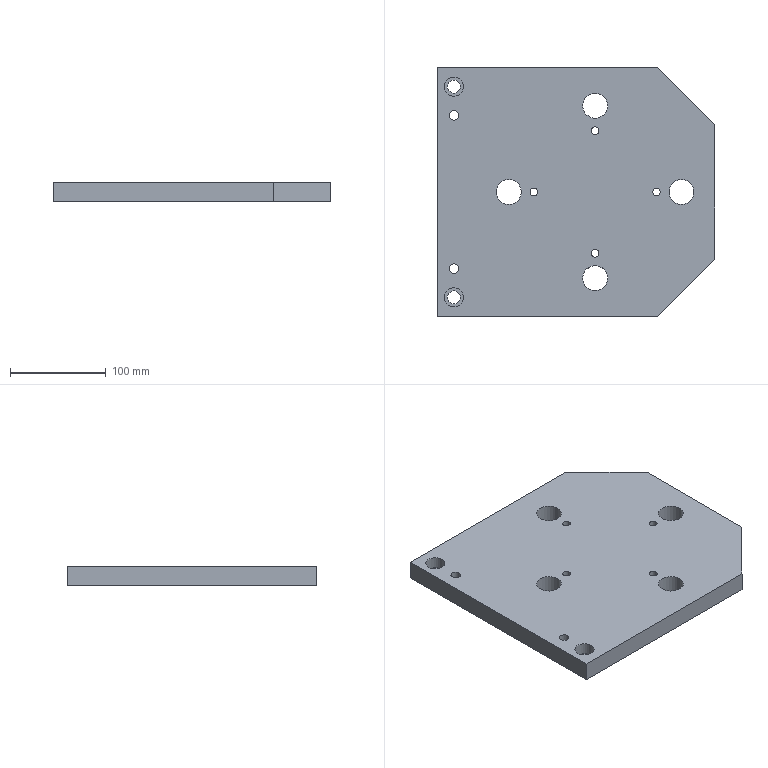Component | NX | DRILL_TEMPLATE | 1 solid | 24 faces | volume 1376259 mm3 | cylinder 14 | plane 10 | commonest cylinder face diameters 26 x4 8 x4 13.5 x2 20 x2 10 x2